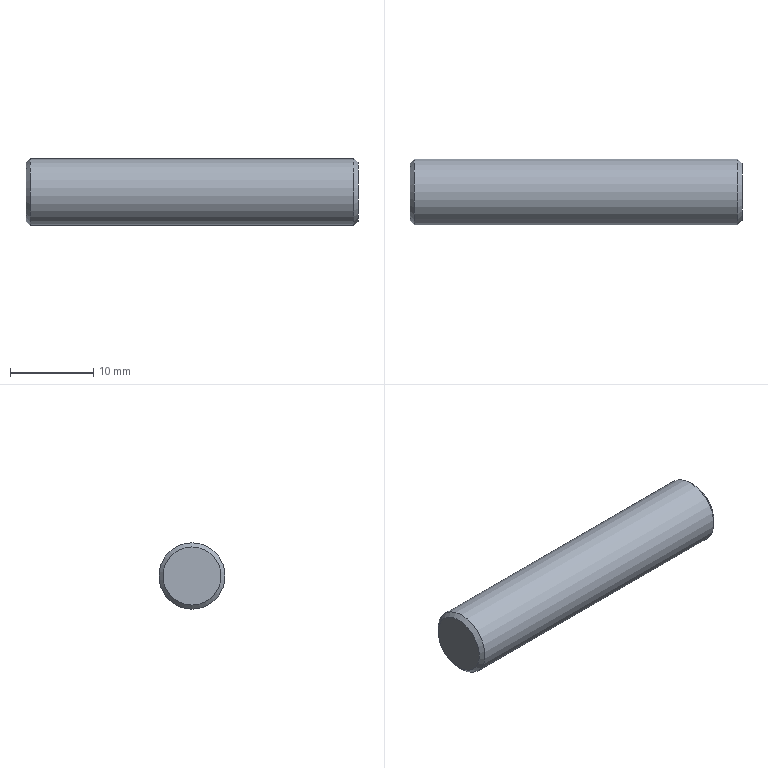Component | NX | DOWEL_PIN_8X40 | 1 solid | 5 faces | box 40 x 8 x 8 mm | volume 2005 mm3 | plane 2 | cone 2 | cylinder 1 | commonest cylinder face diameters 8 x1
STEP:
#1=CARTESIAN_POINT('',(0.,0.,0.));
#2=DIRECTION('',(0.,0.,1.));
#3=DIRECTION('',(1.,0.,0.));
#4=AXIS2_PLACEMENT_3D('',#1,#2,#3);
#5=CARTESIAN_POINT('',(39.511,67.872,-4.));
#6=VERTEX_POINT('',#5);
#7=CARTESIAN_POINT('',(39.511,67.872,-0.));
#8=DIRECTION('',(-1.,0.,0.));
#9=DIRECTION('',(0.,0.,-1.));
#10=AXIS2_PLACEMENT_3D('',#7,#8,#9);
#11=CIRCLE('',#10,4.);
#12=CARTESIAN_POINT('',(20.011,67.872,-0.));
#13=DIRECTION('',(-1.,0.,0.));
#14=DIRECTION('',(0.,0.,1.));
#15=AXIS2_PLACEMENT_3D('',#12,#13,#14);
#16=CYLINDRICAL_SURFACE('',#15,4.);
#17=CARTESIAN_POINT('',(3.142,-19.5));
#18=DIRECTION('',(1.,0.));
#19=VECTOR('',#18,1.);
#20=LINE('',#17,#19);
#21=(GEOMETRIC_REPRESENTATION_CONTEXT(2)PARAMETRIC_REPRESENTATION_CONTEXT()REPRESENTATION_CONTEXT('',''));
#22=DEFINITIONAL_REPRESENTATION('',(#20),#21);
#23=PCURVE('',#16,#22);
#24=CARTESIAN_POINT('',(40.011,67.872,-0.));
#25=DIRECTION('',(-1.,0.,0.));
#26=DIRECTION('',(0.,0.,1.));
#27=AXIS2_PLACEMENT_3D('',#24,#25,#26);
#28=CONICAL_SURFACE('',#27,3.5,0.7854);
#29=CARTESIAN_POINT('',(3.142,0.5));
#30=DIRECTION('',(1.,0.));
#31=VECTOR('',#30,1.);
#32=LINE('',#29,#31);
#33=(GEOMETRIC_REPRESENTATION_CONTEXT(2)PARAMETRIC_REPRESENTATION_CONTEXT()REPRESENTATION_CONTEXT('',''));
#34=DEFINITIONAL_REPRESENTATION('',(#32),#33);
#35=PCURVE('',#28,#34);
#36=SURFACE_CURVE('',#11,(#23,#35),.PCURVE_S1.);
#37=EDGE_CURVE('',#6,#6,#36,.T.);
#38=ORIENTED_EDGE('',*,*,#37,.T.);
#39=CARTESIAN_POINT('',(0.5107,67.872,-4.));
#40=VERTEX_POINT('',#39);
#41=CARTESIAN_POINT('',(39.511,67.872,-4.));
#42=CARTESIAN_POINT('',(0.5107,67.872,-4.));
#43=B_SPLINE_CURVE_WITH_KNOTS('',1,(#41,#42),.UNSPECIFIED.,.F.,.F.,(2,2),(-19.5,19.5),.PIECEWISE_BEZIER_KNOTS.);
#44=CARTESIAN_POINT('',(9.425,0.));
#45=DIRECTION('',(0.,1.));
#46=VECTOR('',#45,1.);
#47=LINE('',#44,#46);
#48=(GEOMETRIC_REPRESENTATION_CONTEXT(2)PARAMETRIC_REPRESENTATION_CONTEXT()REPRESENTATION_CONTEXT('',''));
#49=DEFINITIONAL_REPRESENTATION('',(#47),#48);
#50=PCURVE('',#16,#49);
#51=CARTESIAN_POINT('',(3.142,0.));
#52=DIRECTION('',(0.,1.));
#53=VECTOR('',#52,1.);
#54=LINE('',#51,#53);
#55=(GEOMETRIC_REPRESENTATION_CONTEXT(2)PARAMETRIC_REPRESENTATION_CONTEXT()REPRESENTATION_CONTEXT('',''));
#56=DEFINITIONAL_REPRESENTATION('',(#54),#55);
#57=PCURVE('',#16,#56);
#58=SEAM_CURVE('',#43,(#50,#57),.PCURVE_S1.);
#59=EDGE_CURVE('',#6,#40,#58,.T.);
#60=ORIENTED_EDGE('',*,*,#59,.T.);
#61=CARTESIAN_POINT('',(0.5107,67.872,-0.));
#62=DIRECTION('',(1.,0.,0.));
#63=DIRECTION('',(0.,0.,-1.));
#64=AXIS2_PLACEMENT_3D('',#61,#62,#63);
#65=CIRCLE('',#64,4.);
#66=CARTESIAN_POINT('',(9.425,19.5));
#67=DIRECTION('',(-1.,0.));
#68=VECTOR('',#67,1.);
#69=LINE('',#66,#68);
#70=(GEOMETRIC_REPRESENTATION_CONTEXT(2)PARAMETRIC_REPRESENTATION_CONTEXT()REPRESENTATION_CONTEXT('',''));
#71=DEFINITIONAL_REPRESENTATION('',(#69),#70);
#72=PCURVE('',#16,#71);
#73=CARTESIAN_POINT('',(0.5107,67.872,-0.));
#74=DIRECTION('',(1.,0.,0.));
#75=DIRECTION('',(0.,0.,-1.));
#76=AXIS2_PLACEMENT_3D('',#73,#74,#75);
#77=CONICAL_SURFACE('',#76,4.,0.7854);
#78=CARTESIAN_POINT('',(0.,0.));
#79=DIRECTION('',(1.,0.));
#80=VECTOR('',#79,1.);
#81=LINE('',#78,#80);
#82=(GEOMETRIC_REPRESENTATION_CONTEXT(2)PARAMETRIC_REPRESENTATION_CONTEXT()REPRESENTATION_CONTEXT('',''));
#83=DEFINITIONAL_REPRESENTATION('',(#81),#82);
#84=PCURVE('',#77,#83);
#85=SURFACE_CURVE('',#65,(#72,#84),.PCURVE_S1.);
#86=EDGE_CURVE('',#40,#40,#85,.T.);
#87=ORIENTED_EDGE('',*,*,#86,.T.);
#88=ORIENTED_EDGE('',*,*,#59,.F.);
#89=EDGE_LOOP('',(#38,#60,#87,#88));
#90=FACE_BOUND('',#89,.T.);
#91=ADVANCED_FACE('',(#90),#16,.T.);
#92=CARTESIAN_POINT('',(40.011,67.872,-3.5));
#93=VERTEX_POINT('',#92);
#94=CARTESIAN_POINT('',(40.011,67.872,-0.));
#95=DIRECTION('',(1.,0.,0.));
#96=DIRECTION('',(0.,0.,-1.));
#97=AXIS2_PLACEMENT_3D('',#94,#95,#96);
#98=CIRCLE('',#97,3.5);
#99=CARTESIAN_POINT('',(40.011,67.872,-0.));
#100=DIRECTION('',(1.,0.,0.));
#101=DIRECTION('',(0.,0.,-1.));
#102=AXIS2_PLACEMENT_3D('',#99,#100,#101);
#103=PLANE('',#102);
#104=CARTESIAN_POINT('',(0.,0.));
#105=DIRECTION('',(1.,0.));
#106=AXIS2_PLACEMENT_2D('',#104,#105);
#107=CIRCLE('',#106,3.5);
#108=(GEOMETRIC_REPRESENTATION_CONTEXT(2)PARAMETRIC_REPRESENTATION_CONTEXT()REPRESENTATION_CONTEXT('',''));
#109=DEFINITIONAL_REPRESENTATION('',(#107),#108);
#110=PCURVE('',#103,#109);
#111=CARTESIAN_POINT('',(9.425,0.));
#112=DIRECTION('',(-1.,0.));
#113=VECTOR('',#112,1.);
#114=LINE('',#111,#113);
#115=(GEOMETRIC_REPRESENTATION_CONTEXT(2)PARAMETRIC_REPRESENTATION_CONTEXT()REPRESENTATION_CONTEXT('',''));
#116=DEFINITIONAL_REPRESENTATION('',(#114),#115);
#117=PCURVE('',#28,#116);
#118=SURFACE_CURVE('',#98,(#110,#117),.PCURVE_S1.);
#119=EDGE_CURVE('',#93,#93,#118,.T.);
#120=ORIENTED_EDGE('',*,*,#119,.T.);
#121=EDGE_LOOP('',(#120));
#122=FACE_BOUND('',#121,.T.);
#123=ADVANCED_FACE('',(#122),#103,.T.);
#124=CARTESIAN_POINT('',(0.01066,67.872,-3.5));
#125=VERTEX_POINT('',#124);
#126=CARTESIAN_POINT('',(0.01066,67.872,-0.));
#127=DIRECTION('',(-1.,0.,0.));
#128=DIRECTION('',(0.,0.,-1.));
#129=AXIS2_PLACEMENT_3D('',#126,#127,#128);
#130=CIRCLE('',#129,3.5);
#131=CARTESIAN_POINT('',(0.01066,67.872,-0.));
#132=DIRECTION('',(1.,0.,0.));
#133=DIRECTION('',(0.,0.,-1.));
#134=AXIS2_PLACEMENT_3D('',#131,#132,#133);
#135=PLANE('',#134);
#136=CARTESIAN_POINT('',(3.5,0.));
#137=CARTESIAN_POINT('',(3.5,-6.062));
#138=CARTESIAN_POINT('',(-1.75,-3.031));
#139=CARTESIAN_POINT('',(-7.,-0.));
#140=CARTESIAN_POINT('',(-1.75,3.031));
#141=CARTESIAN_POINT('',(3.5,6.062));
#142=CARTESIAN_POINT('',(3.5,0.));
#143=(BOUNDED_CURVE()B_SPLINE_CURVE(2,(#136,#137,#138,#139,#140,#141,#142),.UNSPECIFIED.,.T.,.F.)B_SPLINE_CURVE_WITH_KNOTS((1,2,2,2,2,1),(-2.094,0.,2.094,4.189,6.283,8.378),.UNSPECIFIED.)CURVE()GEOMETRIC_REPRESENTATION_ITEM()RATIONAL_B_SPLINE_CURVE((1.,0.5,1.,0.5,1.,0.5,1.))REPRESENTATION_ITEM(''));
#144=(GEOMETRIC_REPRESENTATION_CONTEXT(2)PARAMETRIC_REPRESENTATION_CONTEXT()REPRESENTATION_CONTEXT('',''));
#145=DEFINITIONAL_REPRESENTATION('',(#143),#144);
#146=PCURVE('',#135,#145);
#147=CARTESIAN_POINT('',(6.283,-0.5));
#148=DIRECTION('',(-1.,0.));
#149=VECTOR('',#148,1.);
#150=LINE('',#147,#149);
#151=(GEOMETRIC_REPRESENTATION_CONTEXT(2)PARAMETRIC_REPRESENTATION_CONTEXT()REPRESENTATION_CONTEXT('',''));
#152=DEFINITIONAL_REPRESENTATION('',(#150),#151);
#153=PCURVE('',#77,#152);
#154=SURFACE_CURVE('',#130,(#146,#153),.PCURVE_S1.);
#155=EDGE_CURVE('',#125,#125,#154,.T.);
#156=ORIENTED_EDGE('',*,*,#155,.T.);
#157=EDGE_LOOP('',(#156));
#158=FACE_BOUND('',#157,.T.);
#159=ADVANCED_FACE('',(#158),#135,.F.);
#160=ORIENTED_EDGE('',*,*,#37,.F.);
#161=CARTESIAN_POINT('',(40.011,67.872,-3.5));
#162=CARTESIAN_POINT('',(39.511,67.872,-4.));
#163=B_SPLINE_CURVE_WITH_KNOTS('',1,(#161,#162),.UNSPECIFIED.,.F.,.F.,(2,2),(0.,0.7071),.PIECEWISE_BEZIER_KNOTS.);
#164=CARTESIAN_POINT('',(3.142,0.));
#165=DIRECTION('',(0.,1.));
#166=VECTOR('',#165,1.);
#167=LINE('',#164,#166);
#168=(GEOMETRIC_REPRESENTATION_CONTEXT(2)PARAMETRIC_REPRESENTATION_CONTEXT()REPRESENTATION_CONTEXT('',''));
#169=DEFINITIONAL_REPRESENTATION('',(#167),#168);
#170=PCURVE('',#28,#169);
#171=CARTESIAN_POINT('',(9.425,0.));
#172=DIRECTION('',(0.,1.));
#173=VECTOR('',#172,1.);
#174=LINE('',#171,#173);
#175=(GEOMETRIC_REPRESENTATION_CONTEXT(2)PARAMETRIC_REPRESENTATION_CONTEXT()REPRESENTATION_CONTEXT('',''));
#176=DEFINITIONAL_REPRESENTATION('',(#174),#175);
#177=PCURVE('',#28,#176);
#178=SEAM_CURVE('',#163,(#170,#177),.PCURVE_S1.);
#179=EDGE_CURVE('',#93,#6,#178,.T.);
#180=ORIENTED_EDGE('',*,*,#179,.F.);
#181=ORIENTED_EDGE('',*,*,#119,.F.);
#182=ORIENTED_EDGE('',*,*,#179,.T.);
#183=EDGE_LOOP('',(#160,#180,#181,#182));
#184=FACE_BOUND('',#183,.T.);
#185=ADVANCED_FACE('',(#184),#28,.T.);
#186=ORIENTED_EDGE('',*,*,#155,.F.);
#187=CARTESIAN_POINT('',(0.01066,67.872,-3.5));
#188=CARTESIAN_POINT('',(0.5107,67.872,-4.));
#189=B_SPLINE_CURVE_WITH_KNOTS('',1,(#187,#188),.UNSPECIFIED.,.F.,.F.,(2,2),(-0.7071,0.),.PIECEWISE_BEZIER_KNOTS.);
#190=CARTESIAN_POINT('',(6.283,0.));
#191=DIRECTION('',(0.,1.));
#192=VECTOR('',#191,1.);
#193=LINE('',#190,#192);
#194=(GEOMETRIC_REPRESENTATION_CONTEXT(2)PARAMETRIC_REPRESENTATION_CONTEXT()REPRESENTATION_CONTEXT('',''));
#195=DEFINITIONAL_REPRESENTATION('',(#193),#194);
#196=PCURVE('',#77,#195);
#197=CARTESIAN_POINT('',(0.,0.));
#198=DIRECTION('',(0.,1.));
#199=VECTOR('',#198,1.);
#200=LINE('',#197,#199);
#201=(GEOMETRIC_REPRESENTATION_CONTEXT(2)PARAMETRIC_REPRESENTATION_CONTEXT()REPRESENTATION_CONTEXT('',''));
#202=DEFINITIONAL_REPRESENTATION('',(#200),#201);
#203=PCURVE('',#77,#202);
#204=SEAM_CURVE('',#189,(#196,#203),.PCURVE_S1.);
#205=EDGE_CURVE('',#125,#40,#204,.T.);
#206=ORIENTED_EDGE('',*,*,#205,.T.);
#207=ORIENTED_EDGE('',*,*,#86,.F.);
#208=ORIENTED_EDGE('',*,*,#205,.F.);
#209=EDGE_LOOP('',(#186,#206,#207,#208));
#210=FACE_BOUND('',#209,.T.);
#211=ADVANCED_FACE('',(#210),#77,.T.);
#212=CLOSED_SHELL('',(#91,#123,#159,#185,#211));
#213=MANIFOLD_SOLID_BREP('',#212);
#214=(LENGTH_UNIT()NAMED_UNIT(*)SI_UNIT(.MILLI.,.METRE.));
#215=UNCERTAINTY_MEASURE_WITH_UNIT(LENGTH_MEASURE(0.00001),#214,'','');
#216=(NAMED_UNIT(*)PLANE_ANGLE_UNIT()SI_UNIT($,.RADIAN.));
#217=(NAMED_UNIT(*)SI_UNIT($,.STERADIAN.)SOLID_ANGLE_UNIT());
#218=(GEOMETRIC_REPRESENTATION_CONTEXT(3)GLOBAL_UNCERTAINTY_ASSIGNED_CONTEXT((#215))GLOBAL_UNIT_ASSIGNED_CONTEXT((#214,#216,#217))REPRESENTATION_CONTEXT('',''));
#219=ADVANCED_BREP_SHAPE_REPRESENTATION('',(#4,#213),#218);